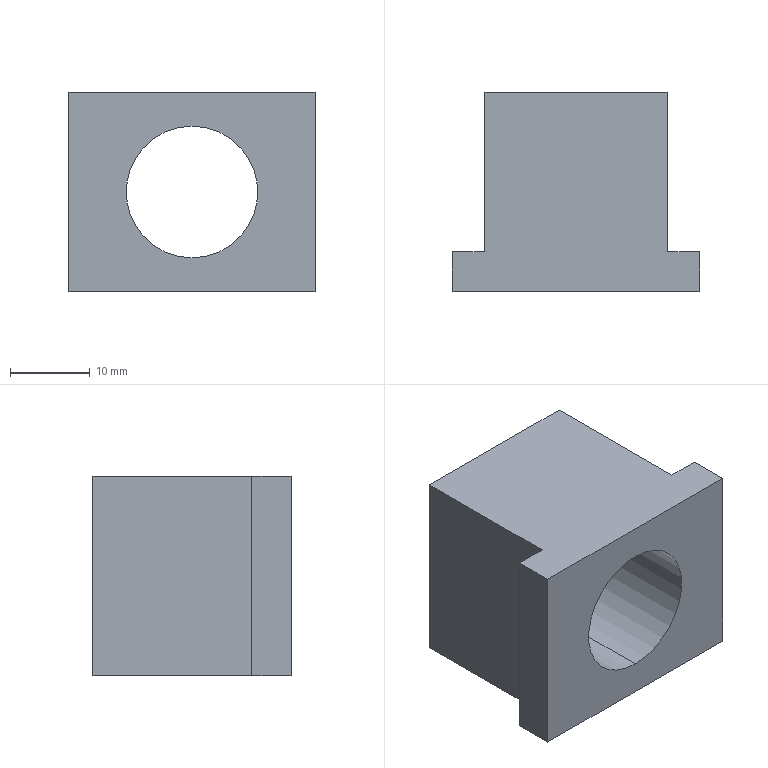Component | SolidWorks | 8TC-A15004-D0-14A-1 | 1 solid | 12 faces | box 31 x 25 x 25 mm | volume 10029 mm3 | plane 10 | cylinder 2 | commonest cylinder face diameters 16.5 x2 | material #45
build123d program:
from build123d import *

# Parameters (mm, degrees)
SKETCH1_W              = 25
SKETCH1_H              = 31
BOSS_EXTRUDE1_DEPTH    = 25
SKETCH2_W              = 20
SKETCH2_H              = 4
CUT_EXTRUDE1_DEPTH     = 39.604
M18X1_5_TAPPED_HOLE1_D = 16.5


with BuildPart() as part:
    # Sketch1 → Boss-Extrude1 (new body)
    with BuildSketch(Plane.XY):
        Rectangle(SKETCH1_W, SKETCH1_H)
    extrude(amount=BOSS_EXTRUDE1_DEPTH)

    # Sketch2 → Cut-Extrude1 (cut, through all)
    with BuildSketch(Plane(origin=(12.5, 0, 0), x_dir=(0, 0, -1), z_dir=(1, 0, 0))):
        with Locations((-15, -13.5)):
            Rectangle(SKETCH2_W, SKETCH2_H)
        with Locations((-15, 13.5)):
            Rectangle(SKETCH2_W, SKETCH2_H)
    extrude(amount=-CUT_EXTRUDE1_DEPTH, mode=Mode.SUBTRACT)

    # M18x1.5 Tapped Hole1 (through all)
    with Locations(Plane.XY.offset(25)):
        with Locations((0, 0)):
            Hole(M18X1_5_TAPPED_HOLE1_D / 2)


solid = part.part

# Placed as in the assembly
solid = solid.moved(Location((-7.5, 353, 0), (-90, 0, 90)))
STEP:
#1=COLOUR_RGB('',0.7922,0.8196,0.9333);
#2=FILL_AREA_STYLE_COLOUR('',#1);
#3=FILL_AREA_STYLE('',(#2));
#4=SURFACE_STYLE_FILL_AREA(#3);
#5=SURFACE_SIDE_STYLE('',(#4));
#6=SURFACE_STYLE_USAGE(.BOTH.,#5);
#7=PRESENTATION_STYLE_ASSIGNMENT((#6));
#8=CARTESIAN_POINT('',(-0.2953,13.898,-0.3248));
#9=VERTEX_POINT('',#8);
#10=CARTESIAN_POINT('',(-0.2953,13.898,0.3248));
#11=VERTEX_POINT('',#10);
#12=CARTESIAN_POINT('',(-0.2953,13.898,-0.));
#13=DIRECTION('',(-0.,1.,0.));
#14=DIRECTION('',(0.,0.,1.));
#15=AXIS2_PLACEMENT_3D('',#12,#13,#14);
#16=CIRCLE('',#15,0.3248);
#17=EDGE_CURVE('',#9,#11,#16,.T.);
#18=ORIENTED_EDGE('',*,*,#17,.F.);
#19=CARTESIAN_POINT('',(-0.2953,14.882,-0.3248));
#20=VERTEX_POINT('',#19);
#21=CARTESIAN_POINT('',(-0.2953,14.882,-0.3248));
#22=DIRECTION('',(-0.,1.,0.));
#23=VECTOR('',#22,39.37);
#24=LINE('',#21,#23);
#25=EDGE_CURVE('',#9,#20,#24,.T.);
#26=ORIENTED_EDGE('',*,*,#25,.T.);
#27=CARTESIAN_POINT('',(-0.2953,14.882,0.3248));
#28=VERTEX_POINT('',#27);
#29=CARTESIAN_POINT('',(-0.2953,14.882,-0.));
#30=DIRECTION('',(-0.,1.,0.));
#31=DIRECTION('',(0.,0.,1.));
#32=AXIS2_PLACEMENT_3D('',#29,#30,#31);
#33=CIRCLE('',#32,0.3248);
#34=EDGE_CURVE('',#20,#28,#33,.T.);
#35=ORIENTED_EDGE('',*,*,#34,.T.);
#36=CARTESIAN_POINT('',(-0.2953,14.882,0.3248));
#37=DIRECTION('',(-0.,1.,0.));
#38=VECTOR('',#37,39.37);
#39=LINE('',#36,#38);
#40=EDGE_CURVE('',#11,#28,#39,.T.);
#41=ORIENTED_EDGE('',*,*,#40,.F.);
#42=EDGE_LOOP('',(#18,#26,#35,#41));
#43=FACE_OUTER_BOUND('',#42,.T.);
#44=CARTESIAN_POINT('',(-0.2953,14.882,-0.));
#45=DIRECTION('',(-0.,1.,0.));
#46=DIRECTION('',(0.,0.,1.));
#47=AXIS2_PLACEMENT_3D('',#44,#45,#46);
#48=CYLINDRICAL_SURFACE('',#47,0.3248);
#49=ADVANCED_FACE('',(#43),#48,.F.);
#50=CARTESIAN_POINT('',(-0.748,14.882,0.4921));
#51=VERTEX_POINT('',#50);
#52=CARTESIAN_POINT('',(0.1575,14.882,0.4921));
#53=VERTEX_POINT('',#52);
#54=CARTESIAN_POINT('',(-0.9055,14.882,0.4921));
#55=DIRECTION('',(1.,0.,0.));
#56=VECTOR('',#55,39.37);
#57=LINE('',#54,#56);
#58=EDGE_CURVE('',#51,#53,#57,.T.);
#59=ORIENTED_EDGE('',*,*,#58,.F.);
#60=CARTESIAN_POINT('',(-0.748,14.094,0.4921));
#61=VERTEX_POINT('',#60);
#62=CARTESIAN_POINT('',(-0.748,14.882,0.4921));
#63=DIRECTION('',(-0.,1.,0.));
#64=VECTOR('',#63,39.37);
#65=LINE('',#62,#64);
#66=EDGE_CURVE('',#61,#51,#65,.T.);
#67=ORIENTED_EDGE('',*,*,#66,.F.);
#68=CARTESIAN_POINT('',(-0.9055,14.094,0.4921));
#69=VERTEX_POINT('',#68);
#70=CARTESIAN_POINT('',(-0.9055,14.094,0.4921));
#71=DIRECTION('',(1.,0.,0.));
#72=VECTOR('',#71,39.37);
#73=LINE('',#70,#72);
#74=EDGE_CURVE('',#69,#61,#73,.T.);
#75=ORIENTED_EDGE('',*,*,#74,.F.);
#76=CARTESIAN_POINT('',(-0.9055,13.898,0.4921));
#77=VERTEX_POINT('',#76);
#78=CARTESIAN_POINT('',(-0.9055,14.882,0.4921));
#79=DIRECTION('',(0.,-1.,-0.));
#80=VECTOR('',#79,39.37);
#81=LINE('',#78,#80);
#82=EDGE_CURVE('',#69,#77,#81,.T.);
#83=ORIENTED_EDGE('',*,*,#82,.T.);
#84=CARTESIAN_POINT('',(0.315,13.898,0.4921));
#85=VERTEX_POINT('',#84);
#86=CARTESIAN_POINT('',(-0.9055,13.898,0.4921));
#87=DIRECTION('',(1.,0.,0.));
#88=VECTOR('',#87,39.37);
#89=LINE('',#86,#88);
#90=EDGE_CURVE('',#77,#85,#89,.T.);
#91=ORIENTED_EDGE('',*,*,#90,.T.);
#92=CARTESIAN_POINT('',(0.315,14.094,0.4921));
#93=VERTEX_POINT('',#92);
#94=CARTESIAN_POINT('',(0.315,14.882,0.4921));
#95=DIRECTION('',(0.,-1.,-0.));
#96=VECTOR('',#95,39.37);
#97=LINE('',#94,#96);
#98=EDGE_CURVE('',#93,#85,#97,.T.);
#99=ORIENTED_EDGE('',*,*,#98,.F.);
#100=CARTESIAN_POINT('',(0.1575,14.094,0.4921));
#101=VERTEX_POINT('',#100);
#102=CARTESIAN_POINT('',(0.315,14.094,0.4921));
#103=DIRECTION('',(1.,-0.,0.));
#104=VECTOR('',#103,39.37);
#105=LINE('',#102,#104);
#106=EDGE_CURVE('',#101,#93,#105,.T.);
#107=ORIENTED_EDGE('',*,*,#106,.F.);
#108=CARTESIAN_POINT('',(0.1575,14.882,0.4921));
#109=DIRECTION('',(0.,-1.,-0.));
#110=VECTOR('',#109,39.37);
#111=LINE('',#108,#110);
#112=EDGE_CURVE('',#53,#101,#111,.T.);
#113=ORIENTED_EDGE('',*,*,#112,.F.);
#114=EDGE_LOOP('',(#59,#67,#75,#83,#91,#99,#107,#113));
#115=FACE_OUTER_BOUND('',#114,.T.);
#116=CARTESIAN_POINT('',(-0.9055,14.882,0.4921));
#117=DIRECTION('',(0.,0.,-1.));
#118=DIRECTION('',(-0.,1.,0.));
#119=AXIS2_PLACEMENT_3D('',#116,#117,#118);
#120=PLANE('',#119);
#121=ADVANCED_FACE('',(#115),#120,.F.);
#122=CARTESIAN_POINT('',(0.315,14.094,-0.4921));
#123=VERTEX_POINT('',#122);
#124=CARTESIAN_POINT('',(0.315,13.898,-0.4921));
#125=VERTEX_POINT('',#124);
#126=CARTESIAN_POINT('',(0.315,14.882,-0.4921));
#127=DIRECTION('',(0.,-1.,-0.));
#128=VECTOR('',#127,39.37);
#129=LINE('',#126,#128);
#130=EDGE_CURVE('',#123,#125,#129,.T.);
#131=ORIENTED_EDGE('',*,*,#130,.F.);
#132=CARTESIAN_POINT('',(0.315,14.094,-0.4921));
#133=DIRECTION('',(-0.,-0.,1.));
#134=VECTOR('',#133,39.37);
#135=LINE('',#132,#134);
#136=EDGE_CURVE('',#123,#93,#135,.T.);
#137=ORIENTED_EDGE('',*,*,#136,.T.);
#138=ORIENTED_EDGE('',*,*,#98,.T.);
#139=CARTESIAN_POINT('',(0.315,13.898,-0.4921));
#140=DIRECTION('',(0.,0.,-1.));
#141=VECTOR('',#140,39.37);
#142=LINE('',#139,#141);
#143=EDGE_CURVE('',#85,#125,#142,.T.);
#144=ORIENTED_EDGE('',*,*,#143,.T.);
#145=EDGE_LOOP('',(#131,#137,#138,#144));
#146=FACE_OUTER_BOUND('',#145,.T.);
#147=CARTESIAN_POINT('',(0.315,14.882,-0.4921));
#148=DIRECTION('',(-1.,-0.,-0.));
#149=DIRECTION('',(0.,-1.,-0.));
#150=AXIS2_PLACEMENT_3D('',#147,#148,#149);
#151=PLANE('',#150);
#152=ADVANCED_FACE('',(#146),#151,.F.);
#153=CARTESIAN_POINT('',(-0.9055,14.094,-0.4921));
#154=VERTEX_POINT('',#153);
#155=CARTESIAN_POINT('',(-0.748,14.094,-0.4921));
#156=VERTEX_POINT('',#155);
#157=CARTESIAN_POINT('',(-0.9055,14.094,-0.4921));
#158=DIRECTION('',(1.,0.,0.));
#159=VECTOR('',#158,39.37);
#160=LINE('',#157,#159);
#161=EDGE_CURVE('',#154,#156,#160,.T.);
#162=ORIENTED_EDGE('',*,*,#161,.T.);
#163=CARTESIAN_POINT('',(-0.748,14.882,-0.4921));
#164=VERTEX_POINT('',#163);
#165=CARTESIAN_POINT('',(-0.748,14.882,-0.4921));
#166=DIRECTION('',(-0.,1.,0.));
#167=VECTOR('',#166,39.37);
#168=LINE('',#165,#167);
#169=EDGE_CURVE('',#156,#164,#168,.T.);
#170=ORIENTED_EDGE('',*,*,#169,.T.);
#171=CARTESIAN_POINT('',(0.1575,14.882,-0.4921));
#172=VERTEX_POINT('',#171);
#173=CARTESIAN_POINT('',(-0.9055,14.882,-0.4921));
#174=DIRECTION('',(-1.,-0.,-0.));
#175=VECTOR('',#174,39.37);
#176=LINE('',#173,#175);
#177=EDGE_CURVE('',#172,#164,#176,.T.);
#178=ORIENTED_EDGE('',*,*,#177,.F.);
#179=CARTESIAN_POINT('',(0.1575,14.094,-0.4921));
#180=VERTEX_POINT('',#179);
#181=CARTESIAN_POINT('',(0.1575,14.882,-0.4921));
#182=DIRECTION('',(0.,-1.,-0.));
#183=VECTOR('',#182,39.37);
#184=LINE('',#181,#183);
#185=EDGE_CURVE('',#172,#180,#184,.T.);
#186=ORIENTED_EDGE('',*,*,#185,.T.);
#187=CARTESIAN_POINT('',(0.315,14.094,-0.4921));
#188=DIRECTION('',(1.,-0.,0.));
#189=VECTOR('',#188,39.37);
#190=LINE('',#187,#189);
#191=EDGE_CURVE('',#180,#123,#190,.T.);
#192=ORIENTED_EDGE('',*,*,#191,.T.);
#193=ORIENTED_EDGE('',*,*,#130,.T.);
#194=CARTESIAN_POINT('',(-0.9055,13.898,-0.4921));
#195=VERTEX_POINT('',#194);
#196=CARTESIAN_POINT('',(-0.9055,13.898,-0.4921));
#197=DIRECTION('',(-1.,-0.,-0.));
#198=VECTOR('',#197,39.37);
#199=LINE('',#196,#198);
#200=EDGE_CURVE('',#125,#195,#199,.T.);
#201=ORIENTED_EDGE('',*,*,#200,.T.);
#202=CARTESIAN_POINT('',(-0.9055,14.882,-0.4921));
#203=DIRECTION('',(0.,-1.,-0.));
#204=VECTOR('',#203,39.37);
#205=LINE('',#202,#204);
#206=EDGE_CURVE('',#154,#195,#205,.T.);
#207=ORIENTED_EDGE('',*,*,#206,.F.);
#208=EDGE_LOOP('',(#162,#170,#178,#186,#192,#193,#201,#207));
#209=FACE_OUTER_BOUND('',#208,.T.);
#210=CARTESIAN_POINT('',(-0.9055,14.882,-0.4921));
#211=DIRECTION('',(-0.,-0.,1.));
#212=DIRECTION('',(0.,-1.,-0.));
#213=AXIS2_PLACEMENT_3D('',#210,#211,#212);
#214=PLANE('',#213);
#215=ADVANCED_FACE('',(#209),#214,.F.);
#216=ORIENTED_EDGE('',*,*,#82,.F.);
#217=CARTESIAN_POINT('',(-0.9055,14.094,-0.4921));
#218=DIRECTION('',(-0.,-0.,1.));
#219=VECTOR('',#218,39.37);
#220=LINE('',#217,#219);
#221=EDGE_CURVE('',#154,#69,#220,.T.);
#222=ORIENTED_EDGE('',*,*,#221,.F.);
#223=ORIENTED_EDGE('',*,*,#206,.T.);
#224=CARTESIAN_POINT('',(-0.9055,13.898,-0.4921));
#225=DIRECTION('',(-0.,-0.,1.));
#226=VECTOR('',#225,39.37);
#227=LINE('',#224,#226);
#228=EDGE_CURVE('',#195,#77,#227,.T.);
#229=ORIENTED_EDGE('',*,*,#228,.T.);
#230=EDGE_LOOP('',(#216,#222,#223,#229));
#231=FACE_OUTER_BOUND('',#230,.T.);
#232=CARTESIAN_POINT('',(-0.9055,14.882,-0.4921));
#233=DIRECTION('',(1.,0.,0.));
#234=DIRECTION('',(-0.,1.,0.));
#235=AXIS2_PLACEMENT_3D('',#232,#233,#234);
#236=PLANE('',#235);
#237=ADVANCED_FACE('',(#231),#236,.F.);
#238=CARTESIAN_POINT('',(-0.2953,14.882,-0.));
#239=DIRECTION('',(-0.,1.,0.));
#240=DIRECTION('',(0.,0.,1.));
#241=AXIS2_PLACEMENT_3D('',#238,#239,#240);
#242=CIRCLE('',#241,0.3248);
#243=EDGE_CURVE('',#28,#20,#242,.T.);
#244=ORIENTED_EDGE('',*,*,#243,.F.);
#245=ORIENTED_EDGE('',*,*,#34,.F.);
#246=EDGE_LOOP('',(#244,#245));
#247=FACE_BOUND('',#246,.T.);
#248=ORIENTED_EDGE('',*,*,#177,.T.);
#249=CARTESIAN_POINT('',(-0.748,14.882,-0.4921));
#250=DIRECTION('',(-0.,-0.,1.));
#251=VECTOR('',#250,39.37);
#252=LINE('',#249,#251);
#253=EDGE_CURVE('',#164,#51,#252,.T.);
#254=ORIENTED_EDGE('',*,*,#253,.T.);
#255=ORIENTED_EDGE('',*,*,#58,.T.);
#256=CARTESIAN_POINT('',(0.1575,14.882,-0.4921));
#257=DIRECTION('',(-0.,-0.,1.));
#258=VECTOR('',#257,39.37);
#259=LINE('',#256,#258);
#260=EDGE_CURVE('',#172,#53,#259,.T.);
#261=ORIENTED_EDGE('',*,*,#260,.F.);
#262=EDGE_LOOP('',(#248,#254,#255,#261));
#263=FACE_OUTER_BOUND('',#262,.T.);
#264=CARTESIAN_POINT('',(-0.2953,14.882,-0.));
#265=DIRECTION('',(0.,-1.,-0.));
#266=DIRECTION('',(0.,0.,-1.));
#267=AXIS2_PLACEMENT_3D('',#264,#265,#266);
#268=PLANE('',#267);
#269=ADVANCED_FACE('',(#247,#263),#268,.F.);
#270=CARTESIAN_POINT('',(-0.2953,13.898,-0.));
#271=DIRECTION('',(-0.,1.,0.));
#272=DIRECTION('',(0.,0.,1.));
#273=AXIS2_PLACEMENT_3D('',#270,#271,#272);
#274=CIRCLE('',#273,0.3248);
#275=EDGE_CURVE('',#11,#9,#274,.T.);
#276=ORIENTED_EDGE('',*,*,#275,.T.);
#277=ORIENTED_EDGE('',*,*,#17,.T.);
#278=EDGE_LOOP('',(#276,#277));
#279=FACE_BOUND('',#278,.T.);
#280=ORIENTED_EDGE('',*,*,#90,.F.);
#281=ORIENTED_EDGE('',*,*,#228,.F.);
#282=ORIENTED_EDGE('',*,*,#200,.F.);
#283=ORIENTED_EDGE('',*,*,#143,.F.);
#284=EDGE_LOOP('',(#280,#281,#282,#283));
#285=FACE_OUTER_BOUND('',#284,.T.);
#286=CARTESIAN_POINT('',(-0.2953,13.898,-0.));
#287=DIRECTION('',(0.,-1.,-0.));
#288=DIRECTION('',(0.,0.,-1.));
#289=AXIS2_PLACEMENT_3D('',#286,#287,#288);
#290=PLANE('',#289);
#291=ADVANCED_FACE('',(#279,#285),#290,.T.);
#292=ORIENTED_EDGE('',*,*,#106,.T.);
#293=ORIENTED_EDGE('',*,*,#136,.F.);
#294=ORIENTED_EDGE('',*,*,#191,.F.);
#295=CARTESIAN_POINT('',(0.1575,14.094,-0.4921));
#296=DIRECTION('',(-0.,-0.,1.));
#297=VECTOR('',#296,39.37);
#298=LINE('',#295,#297);
#299=EDGE_CURVE('',#180,#101,#298,.T.);
#300=ORIENTED_EDGE('',*,*,#299,.T.);
#301=EDGE_LOOP('',(#292,#293,#294,#300));
#302=FACE_OUTER_BOUND('',#301,.T.);
#303=CARTESIAN_POINT('',(0.315,14.094,-0.4921));
#304=DIRECTION('',(-0.,-1.,-0.));
#305=DIRECTION('',(1.,-0.,0.));
#306=AXIS2_PLACEMENT_3D('',#303,#304,#305);
#307=PLANE('',#306);
#308=ADVANCED_FACE('',(#302),#307,.F.);
#309=ORIENTED_EDGE('',*,*,#112,.T.);
#310=ORIENTED_EDGE('',*,*,#299,.F.);
#311=ORIENTED_EDGE('',*,*,#185,.F.);
#312=ORIENTED_EDGE('',*,*,#260,.T.);
#313=EDGE_LOOP('',(#309,#310,#311,#312));
#314=FACE_OUTER_BOUND('',#313,.T.);
#315=CARTESIAN_POINT('',(0.1575,14.882,-0.4921));
#316=DIRECTION('',(-1.,-0.,-0.));
#317=DIRECTION('',(0.,-1.,-0.));
#318=AXIS2_PLACEMENT_3D('',#315,#316,#317);
#319=PLANE('',#318);
#320=ADVANCED_FACE('',(#314),#319,.F.);
#321=ORIENTED_EDGE('',*,*,#66,.T.);
#322=ORIENTED_EDGE('',*,*,#253,.F.);
#323=ORIENTED_EDGE('',*,*,#169,.F.);
#324=CARTESIAN_POINT('',(-0.748,14.094,-0.4921));
#325=DIRECTION('',(-0.,-0.,1.));
#326=VECTOR('',#325,39.37);
#327=LINE('',#324,#326);
#328=EDGE_CURVE('',#156,#61,#327,.T.);
#329=ORIENTED_EDGE('',*,*,#328,.T.);
#330=EDGE_LOOP('',(#321,#322,#323,#329));
#331=FACE_OUTER_BOUND('',#330,.T.);
#332=CARTESIAN_POINT('',(-0.748,14.882,-0.4921));
#333=DIRECTION('',(1.,0.,0.));
#334=DIRECTION('',(-0.,1.,0.));
#335=AXIS2_PLACEMENT_3D('',#332,#333,#334);
#336=PLANE('',#335);
#337=ADVANCED_FACE('',(#331),#336,.F.);
#338=ORIENTED_EDGE('',*,*,#74,.T.);
#339=ORIENTED_EDGE('',*,*,#328,.F.);
#340=ORIENTED_EDGE('',*,*,#161,.F.);
#341=ORIENTED_EDGE('',*,*,#221,.T.);
#342=EDGE_LOOP('',(#338,#339,#340,#341));
#343=FACE_OUTER_BOUND('',#342,.T.);
#344=CARTESIAN_POINT('',(-0.9055,14.094,-0.4921));
#345=DIRECTION('',(0.,-1.,-0.));
#346=DIRECTION('',(1.,0.,0.));
#347=AXIS2_PLACEMENT_3D('',#344,#345,#346);
#348=PLANE('',#347);
#349=ADVANCED_FACE('',(#343),#348,.F.);
#350=ORIENTED_EDGE('',*,*,#25,.F.);
#351=ORIENTED_EDGE('',*,*,#275,.F.);
#352=ORIENTED_EDGE('',*,*,#40,.T.);
#353=ORIENTED_EDGE('',*,*,#243,.T.);
#354=EDGE_LOOP('',(#350,#351,#352,#353));
#355=FACE_OUTER_BOUND('',#354,.T.);
#356=CARTESIAN_POINT('',(-0.2953,14.882,-0.));
#357=DIRECTION('',(-0.,1.,0.));
#358=DIRECTION('',(0.,0.,1.));
#359=AXIS2_PLACEMENT_3D('',#356,#357,#358);
#360=CYLINDRICAL_SURFACE('',#359,0.3248);
#361=ADVANCED_FACE('',(#355),#360,.F.);
#362=CLOSED_SHELL('',(#49,#121,#152,#215,#237,#269,#291,#308,#320,#337,#349,#361));
#363=MANIFOLD_SOLID_BREP('',#362);
#364=STYLED_ITEM('',(#7),#363);
#365=PRESENTATION_LAYER_ASSIGNMENT('','',(#364));
#366=(LENGTH_UNIT()NAMED_UNIT(*)SI_UNIT($,.METRE.));
#367=LENGTH_MEASURE_WITH_UNIT(LENGTH_MEASURE(0.0254),#366);
#368=DIMENSIONAL_EXPONENTS(1.,0.,0.,0.,0.,0.,0.);
#369=(CONVERSION_BASED_UNIT('',#367)LENGTH_UNIT()NAMED_UNIT(#368));
#370=UNCERTAINTY_MEASURE_WITH_UNIT(LENGTH_MEASURE(0.00001),#369,'','');
#371=(NAMED_UNIT(*)PLANE_ANGLE_UNIT()SI_UNIT($,.RADIAN.));
#372=(NAMED_UNIT(*)SI_UNIT($,.STERADIAN.)SOLID_ANGLE_UNIT());
#373=(GEOMETRIC_REPRESENTATION_CONTEXT(3)GLOBAL_UNCERTAINTY_ASSIGNED_CONTEXT((#370))GLOBAL_UNIT_ASSIGNED_CONTEXT((#369,#371,#372))REPRESENTATION_CONTEXT('',''));
#374=MECHANICAL_DESIGN_GEOMETRIC_PRESENTATION_REPRESENTATION('',(#364),#373);
#375=CARTESIAN_POINT('',(0.,0.,0.));
#376=DIRECTION('',(0.,0.,1.));
#377=DIRECTION('',(1.,0.,0.));
#378=AXIS2_PLACEMENT_3D('',#375,#376,#377);
#379=(LENGTH_UNIT()NAMED_UNIT(*)SI_UNIT($,.METRE.));
#380=LENGTH_MEASURE_WITH_UNIT(LENGTH_MEASURE(0.0254),#379);
#381=DIMENSIONAL_EXPONENTS(1.,0.,0.,0.,0.,0.,0.);
#382=(CONVERSION_BASED_UNIT('',#380)LENGTH_UNIT()NAMED_UNIT(#381));
#383=UNCERTAINTY_MEASURE_WITH_UNIT(LENGTH_MEASURE(0.00001),#382,'','');
#384=(NAMED_UNIT(*)PLANE_ANGLE_UNIT()SI_UNIT($,.RADIAN.));
#385=(NAMED_UNIT(*)SI_UNIT($,.STERADIAN.)SOLID_ANGLE_UNIT());
#386=(GEOMETRIC_REPRESENTATION_CONTEXT(3)GLOBAL_UNCERTAINTY_ASSIGNED_CONTEXT((#383))GLOBAL_UNIT_ASSIGNED_CONTEXT((#382,#384,#385))REPRESENTATION_CONTEXT('',''));
#387=ADVANCED_BREP_SHAPE_REPRESENTATION('',(#363,#378),#386);